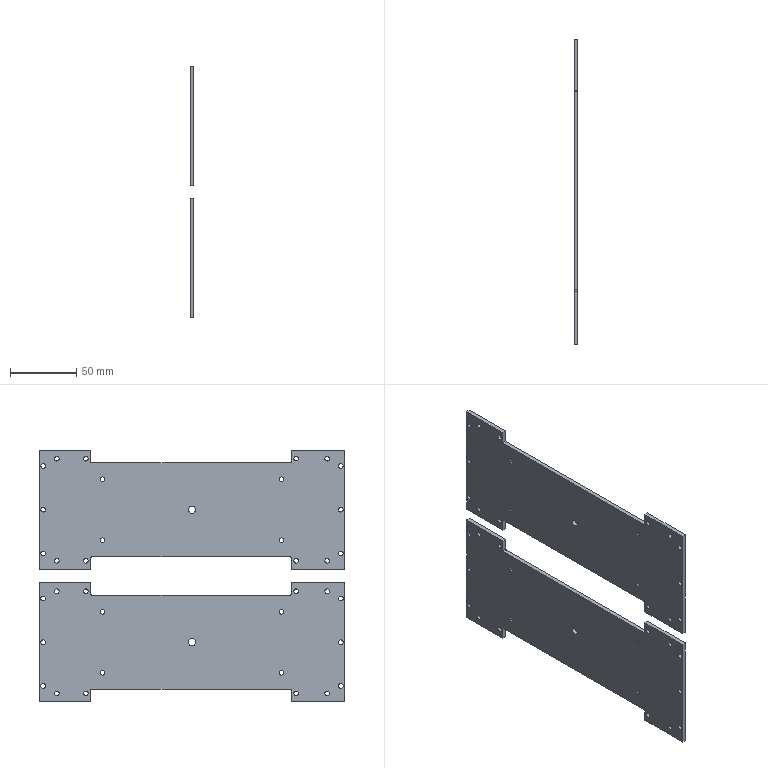CAM job | Mastercam | mm | 5 operations | part box 3 x 230.5 x 190
1. Contour (Ramp) | 4 - 4 平铣刀
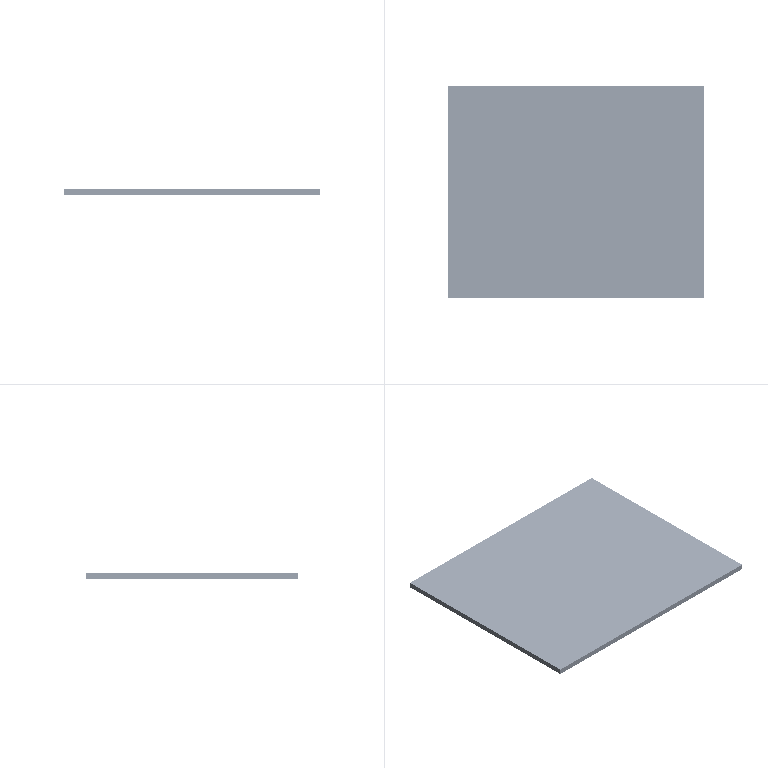2. Contour (Remachining) | 2 - 2 平铣刀
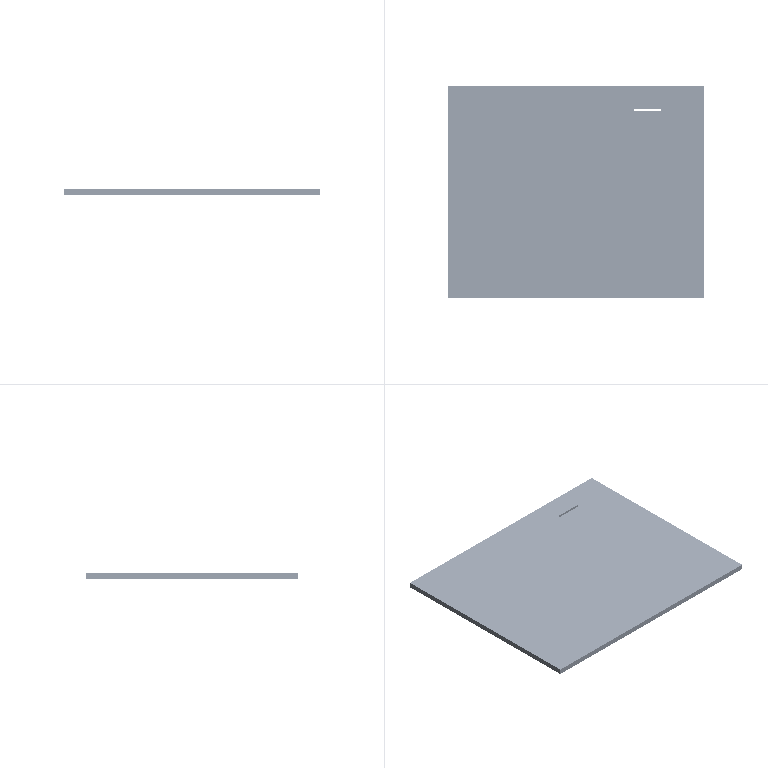3. Contour (2D) | 2 - 2 平铣刀
4. Drill/Counterbore | 5 - 4 倒角刀
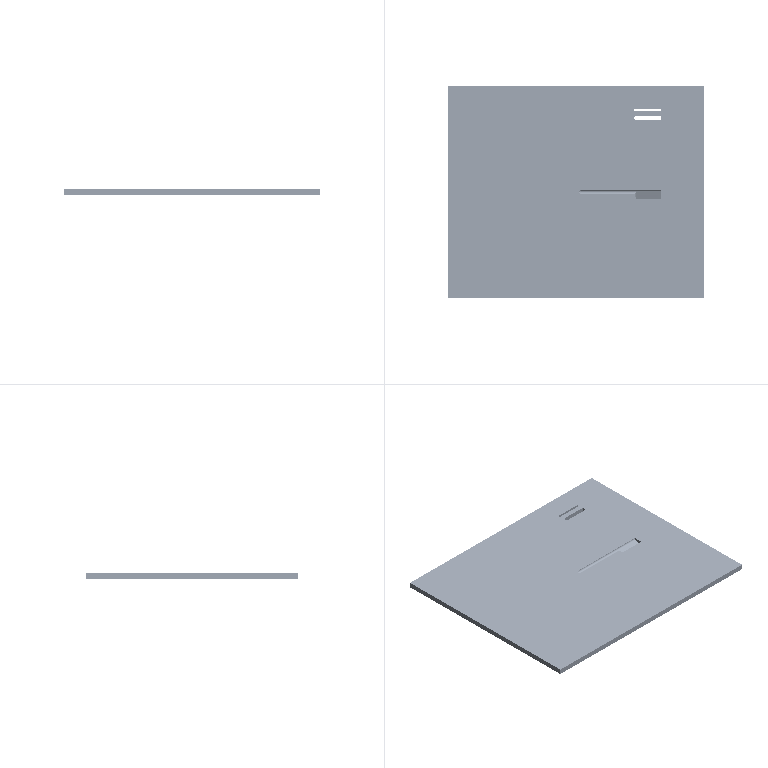5. Contour (2D chamfer) | 5 - 4 倒角刀